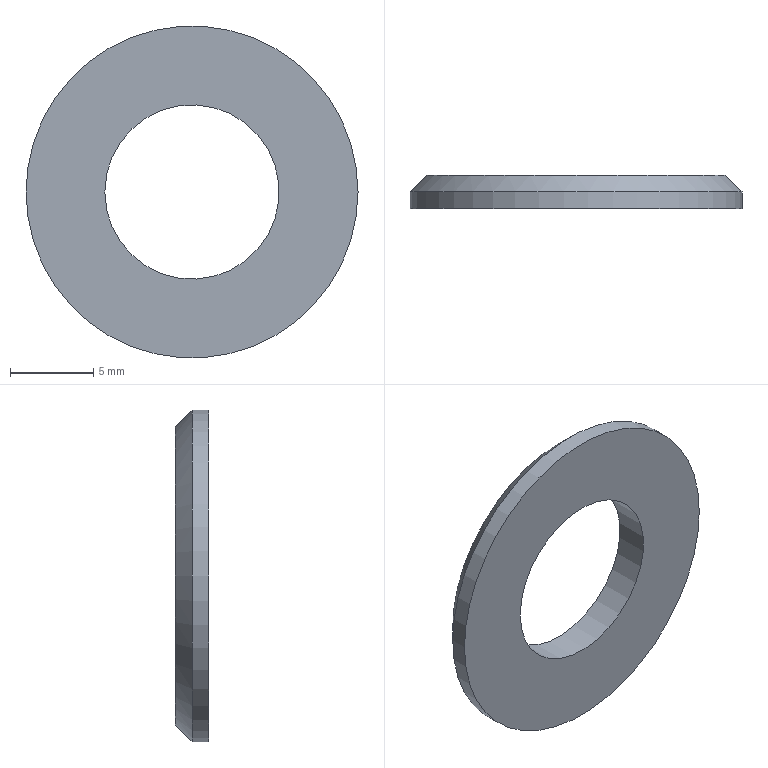Component | NX | GB-T97_2-2002_M10 | 1 solid | 5 faces | box 20 x 2 x 20 mm | volume 425 mm3 | cylinder 2 | plane 2 | cone 1 | commonest cylinder face diameters 20 x1 10.5 x1
STEP:
#1=CARTESIAN_POINT('',(0.,0.,0.));
#2=DIRECTION('',(0.,0.,1.));
#3=DIRECTION('',(1.,0.,0.));
#4=AXIS2_PLACEMENT_3D('',#1,#2,#3);
#5=CARTESIAN_POINT('',(-10.,55.,43.));
#6=VERTEX_POINT('',#5);
#7=CARTESIAN_POINT('',(-0.,55.,43.));
#8=DIRECTION('',(0.,-1.,0.));
#9=DIRECTION('',(-1.,0.,0.));
#10=AXIS2_PLACEMENT_3D('',#7,#8,#9);
#11=CIRCLE('',#10,10.);
#12=CARTESIAN_POINT('',(-0.,56.,43.));
#13=DIRECTION('',(0.,-1.,0.));
#14=DIRECTION('',(1.,0.,0.));
#15=AXIS2_PLACEMENT_3D('',#12,#13,#14);
#16=CYLINDRICAL_SURFACE('',#15,10.);
#17=CARTESIAN_POINT('',(3.142,1.));
#18=DIRECTION('',(1.,0.));
#19=VECTOR('',#18,1.);
#20=LINE('',#17,#19);
#21=(GEOMETRIC_REPRESENTATION_CONTEXT(2)PARAMETRIC_REPRESENTATION_CONTEXT()REPRESENTATION_CONTEXT('',''));
#22=DEFINITIONAL_REPRESENTATION('',(#20),#21);
#23=PCURVE('',#16,#22);
#24=CARTESIAN_POINT('',(-0.,56.,43.));
#25=DIRECTION('',(0.,-1.,0.));
#26=DIRECTION('',(1.,0.,0.));
#27=AXIS2_PLACEMENT_3D('',#24,#25,#26);
#28=CONICAL_SURFACE('',#27,9.,0.7854);
#29=CARTESIAN_POINT('',(3.142,1.));
#30=DIRECTION('',(1.,0.));
#31=VECTOR('',#30,1.);
#32=LINE('',#29,#31);
#33=(GEOMETRIC_REPRESENTATION_CONTEXT(2)PARAMETRIC_REPRESENTATION_CONTEXT()REPRESENTATION_CONTEXT('',''));
#34=DEFINITIONAL_REPRESENTATION('',(#32),#33);
#35=PCURVE('',#28,#34);
#36=SURFACE_CURVE('',#11,(#23,#35),.PCURVE_S1.);
#37=EDGE_CURVE('',#6,#6,#36,.T.);
#38=ORIENTED_EDGE('',*,*,#37,.T.);
#39=CARTESIAN_POINT('',(-10.,54.,43.));
#40=VERTEX_POINT('',#39);
#41=CARTESIAN_POINT('',(-10.,55.,43.));
#42=CARTESIAN_POINT('',(-10.,54.,43.));
#43=B_SPLINE_CURVE_WITH_KNOTS('',1,(#41,#42),.UNSPECIFIED.,.F.,.F.,(2,2),(1.,2.),.PIECEWISE_BEZIER_KNOTS.);
#44=CARTESIAN_POINT('',(9.425,0.));
#45=DIRECTION('',(0.,1.));
#46=VECTOR('',#45,1.);
#47=LINE('',#44,#46);
#48=(GEOMETRIC_REPRESENTATION_CONTEXT(2)PARAMETRIC_REPRESENTATION_CONTEXT()REPRESENTATION_CONTEXT('',''));
#49=DEFINITIONAL_REPRESENTATION('',(#47),#48);
#50=PCURVE('',#16,#49);
#51=CARTESIAN_POINT('',(3.142,0.));
#52=DIRECTION('',(0.,1.));
#53=VECTOR('',#52,1.);
#54=LINE('',#51,#53);
#55=(GEOMETRIC_REPRESENTATION_CONTEXT(2)PARAMETRIC_REPRESENTATION_CONTEXT()REPRESENTATION_CONTEXT('',''));
#56=DEFINITIONAL_REPRESENTATION('',(#54),#55);
#57=PCURVE('',#16,#56);
#58=SEAM_CURVE('',#43,(#50,#57),.PCURVE_S1.);
#59=EDGE_CURVE('',#6,#40,#58,.T.);
#60=ORIENTED_EDGE('',*,*,#59,.T.);
#61=CARTESIAN_POINT('',(-0.,54.,43.));
#62=DIRECTION('',(0.,1.,0.));
#63=DIRECTION('',(-1.,0.,0.));
#64=AXIS2_PLACEMENT_3D('',#61,#62,#63);
#65=CIRCLE('',#64,10.);
#66=CARTESIAN_POINT('',(9.425,2.));
#67=DIRECTION('',(-1.,0.));
#68=VECTOR('',#67,1.);
#69=LINE('',#66,#68);
#70=(GEOMETRIC_REPRESENTATION_CONTEXT(2)PARAMETRIC_REPRESENTATION_CONTEXT()REPRESENTATION_CONTEXT('',''));
#71=DEFINITIONAL_REPRESENTATION('',(#69),#70);
#72=PCURVE('',#16,#71);
#73=CARTESIAN_POINT('',(-0.,54.,43.));
#74=DIRECTION('',(0.,1.,0.));
#75=DIRECTION('',(-1.,0.,0.));
#76=AXIS2_PLACEMENT_3D('',#73,#74,#75);
#77=PLANE('',#76);
#78=CARTESIAN_POINT('',(0.,0.));
#79=DIRECTION('',(1.,0.));
#80=AXIS2_PLACEMENT_2D('',#78,#79);
#81=CIRCLE('',#80,10.);
#82=(GEOMETRIC_REPRESENTATION_CONTEXT(2)PARAMETRIC_REPRESENTATION_CONTEXT()REPRESENTATION_CONTEXT('',''));
#83=DEFINITIONAL_REPRESENTATION('',(#81),#82);
#84=PCURVE('',#77,#83);
#85=SURFACE_CURVE('',#65,(#72,#84),.PCURVE_S1.);
#86=EDGE_CURVE('',#40,#40,#85,.T.);
#87=ORIENTED_EDGE('',*,*,#86,.T.);
#88=ORIENTED_EDGE('',*,*,#59,.F.);
#89=EDGE_LOOP('',(#38,#60,#87,#88));
#90=FACE_BOUND('',#89,.T.);
#91=ADVANCED_FACE('',(#90),#16,.T.);
#92=CARTESIAN_POINT('',(-5.25,56.,43.));
#93=VERTEX_POINT('',#92);
#94=CARTESIAN_POINT('',(-0.,56.,43.));
#95=DIRECTION('',(0.,1.,0.));
#96=DIRECTION('',(-1.,0.,0.));
#97=AXIS2_PLACEMENT_3D('',#94,#95,#96);
#98=CIRCLE('',#97,5.25);
#99=CARTESIAN_POINT('',(-0.,56.,43.));
#100=DIRECTION('',(0.,-1.,0.));
#101=DIRECTION('',(1.,0.,0.));
#102=AXIS2_PLACEMENT_3D('',#99,#100,#101);
#103=CYLINDRICAL_SURFACE('',#102,5.25);
#104=CARTESIAN_POINT('',(9.425,0.));
#105=DIRECTION('',(-1.,0.));
#106=VECTOR('',#105,1.);
#107=LINE('',#104,#106);
#108=(GEOMETRIC_REPRESENTATION_CONTEXT(2)PARAMETRIC_REPRESENTATION_CONTEXT()REPRESENTATION_CONTEXT('',''));
#109=DEFINITIONAL_REPRESENTATION('',(#107),#108);
#110=PCURVE('',#103,#109);
#111=CARTESIAN_POINT('',(-0.,56.,43.));
#112=DIRECTION('',(0.,1.,0.));
#113=DIRECTION('',(-1.,0.,0.));
#114=AXIS2_PLACEMENT_3D('',#111,#112,#113);
#115=PLANE('',#114);
#116=CARTESIAN_POINT('',(0.,0.));
#117=DIRECTION('',(1.,0.));
#118=AXIS2_PLACEMENT_2D('',#116,#117);
#119=CIRCLE('',#118,5.25);
#120=(GEOMETRIC_REPRESENTATION_CONTEXT(2)PARAMETRIC_REPRESENTATION_CONTEXT()REPRESENTATION_CONTEXT('',''));
#121=DEFINITIONAL_REPRESENTATION('',(#119),#120);
#122=PCURVE('',#115,#121);
#123=SURFACE_CURVE('',#98,(#110,#122),.PCURVE_S1.);
#124=EDGE_CURVE('',#93,#93,#123,.T.);
#125=ORIENTED_EDGE('',*,*,#124,.F.);
#126=CARTESIAN_POINT('',(-5.25,54.,43.));
#127=VERTEX_POINT('',#126);
#128=CARTESIAN_POINT('',(-5.25,56.,43.));
#129=CARTESIAN_POINT('',(-5.25,54.,43.));
#130=B_SPLINE_CURVE_WITH_KNOTS('',1,(#128,#129),.UNSPECIFIED.,.F.,.F.,(2,2),(0.,2.),.PIECEWISE_BEZIER_KNOTS.);
#131=CARTESIAN_POINT('',(9.425,0.));
#132=DIRECTION('',(0.,1.));
#133=VECTOR('',#132,1.);
#134=LINE('',#131,#133);
#135=(GEOMETRIC_REPRESENTATION_CONTEXT(2)PARAMETRIC_REPRESENTATION_CONTEXT()REPRESENTATION_CONTEXT('',''));
#136=DEFINITIONAL_REPRESENTATION('',(#134),#135);
#137=PCURVE('',#103,#136);
#138=CARTESIAN_POINT('',(3.142,0.));
#139=DIRECTION('',(0.,1.));
#140=VECTOR('',#139,1.);
#141=LINE('',#138,#140);
#142=(GEOMETRIC_REPRESENTATION_CONTEXT(2)PARAMETRIC_REPRESENTATION_CONTEXT()REPRESENTATION_CONTEXT('',''));
#143=DEFINITIONAL_REPRESENTATION('',(#141),#142);
#144=PCURVE('',#103,#143);
#145=SEAM_CURVE('',#130,(#137,#144),.PCURVE_S1.);
#146=EDGE_CURVE('',#93,#127,#145,.T.);
#147=ORIENTED_EDGE('',*,*,#146,.T.);
#148=CARTESIAN_POINT('',(-0.,54.,43.));
#149=DIRECTION('',(0.,1.,0.));
#150=DIRECTION('',(-1.,0.,0.));
#151=AXIS2_PLACEMENT_3D('',#148,#149,#150);
#152=CIRCLE('',#151,5.25);
#153=CARTESIAN_POINT('',(9.425,2.));
#154=DIRECTION('',(-1.,0.));
#155=VECTOR('',#154,1.);
#156=LINE('',#153,#155);
#157=(GEOMETRIC_REPRESENTATION_CONTEXT(2)PARAMETRIC_REPRESENTATION_CONTEXT()REPRESENTATION_CONTEXT('',''));
#158=DEFINITIONAL_REPRESENTATION('',(#156),#157);
#159=PCURVE('',#103,#158);
#160=CARTESIAN_POINT('',(0.,0.));
#161=DIRECTION('',(1.,0.));
#162=AXIS2_PLACEMENT_2D('',#160,#161);
#163=CIRCLE('',#162,5.25);
#164=(GEOMETRIC_REPRESENTATION_CONTEXT(2)PARAMETRIC_REPRESENTATION_CONTEXT()REPRESENTATION_CONTEXT('',''));
#165=DEFINITIONAL_REPRESENTATION('',(#163),#164);
#166=PCURVE('',#77,#165);
#167=SURFACE_CURVE('',#152,(#159,#166),.PCURVE_S1.);
#168=EDGE_CURVE('',#127,#127,#167,.T.);
#169=ORIENTED_EDGE('',*,*,#168,.T.);
#170=ORIENTED_EDGE('',*,*,#146,.F.);
#171=EDGE_LOOP('',(#125,#147,#169,#170));
#172=FACE_BOUND('',#171,.F.);
#173=ADVANCED_FACE('',(#172),#103,.F.);
#174=CARTESIAN_POINT('',(-9.,56.,43.));
#175=VERTEX_POINT('',#174);
#176=CARTESIAN_POINT('',(-0.,56.,43.));
#177=DIRECTION('',(0.,1.,0.));
#178=DIRECTION('',(-1.,0.,0.));
#179=AXIS2_PLACEMENT_3D('',#176,#177,#178);
#180=CIRCLE('',#179,9.);
#181=CARTESIAN_POINT('',(0.,0.));
#182=DIRECTION('',(1.,0.));
#183=AXIS2_PLACEMENT_2D('',#181,#182);
#184=CIRCLE('',#183,9.);
#185=(GEOMETRIC_REPRESENTATION_CONTEXT(2)PARAMETRIC_REPRESENTATION_CONTEXT()REPRESENTATION_CONTEXT('',''));
#186=DEFINITIONAL_REPRESENTATION('',(#184),#185);
#187=PCURVE('',#115,#186);
#188=CARTESIAN_POINT('',(9.425,0.));
#189=DIRECTION('',(-1.,0.));
#190=VECTOR('',#189,1.);
#191=LINE('',#188,#190);
#192=(GEOMETRIC_REPRESENTATION_CONTEXT(2)PARAMETRIC_REPRESENTATION_CONTEXT()REPRESENTATION_CONTEXT('',''));
#193=DEFINITIONAL_REPRESENTATION('',(#191),#192);
#194=PCURVE('',#28,#193);
#195=SURFACE_CURVE('',#180,(#187,#194),.PCURVE_S1.);
#196=EDGE_CURVE('',#175,#175,#195,.T.);
#197=ORIENTED_EDGE('',*,*,#196,.T.);
#198=EDGE_LOOP('',(#197));
#199=FACE_BOUND('',#198,.T.);
#200=ORIENTED_EDGE('',*,*,#124,.F.);
#201=EDGE_LOOP('',(#200));
#202=FACE_BOUND('',#201,.T.);
#203=ADVANCED_FACE('',(#199,#202),#115,.T.);
#204=ORIENTED_EDGE('',*,*,#86,.F.);
#205=EDGE_LOOP('',(#204));
#206=FACE_BOUND('',#205,.T.);
#207=ORIENTED_EDGE('',*,*,#168,.T.);
#208=EDGE_LOOP('',(#207));
#209=FACE_BOUND('',#208,.T.);
#210=ADVANCED_FACE('',(#206,#209),#77,.F.);
#211=ORIENTED_EDGE('',*,*,#37,.F.);
#212=CARTESIAN_POINT('',(-9.,56.,43.));
#213=CARTESIAN_POINT('',(-10.,55.,43.));
#214=B_SPLINE_CURVE_WITH_KNOTS('',1,(#212,#213),.UNSPECIFIED.,.F.,.F.,(2,2),(0.,1.414),.PIECEWISE_BEZIER_KNOTS.);
#215=CARTESIAN_POINT('',(3.142,0.));
#216=DIRECTION('',(0.,1.));
#217=VECTOR('',#216,1.);
#218=LINE('',#215,#217);
#219=(GEOMETRIC_REPRESENTATION_CONTEXT(2)PARAMETRIC_REPRESENTATION_CONTEXT()REPRESENTATION_CONTEXT('',''));
#220=DEFINITIONAL_REPRESENTATION('',(#218),#219);
#221=PCURVE('',#28,#220);
#222=CARTESIAN_POINT('',(9.425,0.));
#223=DIRECTION('',(0.,1.));
#224=VECTOR('',#223,1.);
#225=LINE('',#222,#224);
#226=(GEOMETRIC_REPRESENTATION_CONTEXT(2)PARAMETRIC_REPRESENTATION_CONTEXT()REPRESENTATION_CONTEXT('',''));
#227=DEFINITIONAL_REPRESENTATION('',(#225),#226);
#228=PCURVE('',#28,#227);
#229=SEAM_CURVE('',#214,(#221,#228),.PCURVE_S1.);
#230=EDGE_CURVE('',#175,#6,#229,.T.);
#231=ORIENTED_EDGE('',*,*,#230,.F.);
#232=ORIENTED_EDGE('',*,*,#196,.F.);
#233=ORIENTED_EDGE('',*,*,#230,.T.);
#234=EDGE_LOOP('',(#211,#231,#232,#233));
#235=FACE_BOUND('',#234,.T.);
#236=ADVANCED_FACE('',(#235),#28,.T.);
#237=CLOSED_SHELL('',(#91,#173,#203,#210,#236));
#238=MANIFOLD_SOLID_BREP('',#237);
#239=(LENGTH_UNIT()NAMED_UNIT(*)SI_UNIT(.MILLI.,.METRE.));
#240=UNCERTAINTY_MEASURE_WITH_UNIT(LENGTH_MEASURE(0.00001),#239,'','');
#241=(NAMED_UNIT(*)PLANE_ANGLE_UNIT()SI_UNIT($,.RADIAN.));
#242=(NAMED_UNIT(*)SI_UNIT($,.STERADIAN.)SOLID_ANGLE_UNIT());
#243=(GEOMETRIC_REPRESENTATION_CONTEXT(3)GLOBAL_UNCERTAINTY_ASSIGNED_CONTEXT((#240))GLOBAL_UNIT_ASSIGNED_CONTEXT((#239,#241,#242))REPRESENTATION_CONTEXT('',''));
#244=ADVANCED_BREP_SHAPE_REPRESENTATION('',(#4,#238),#243);